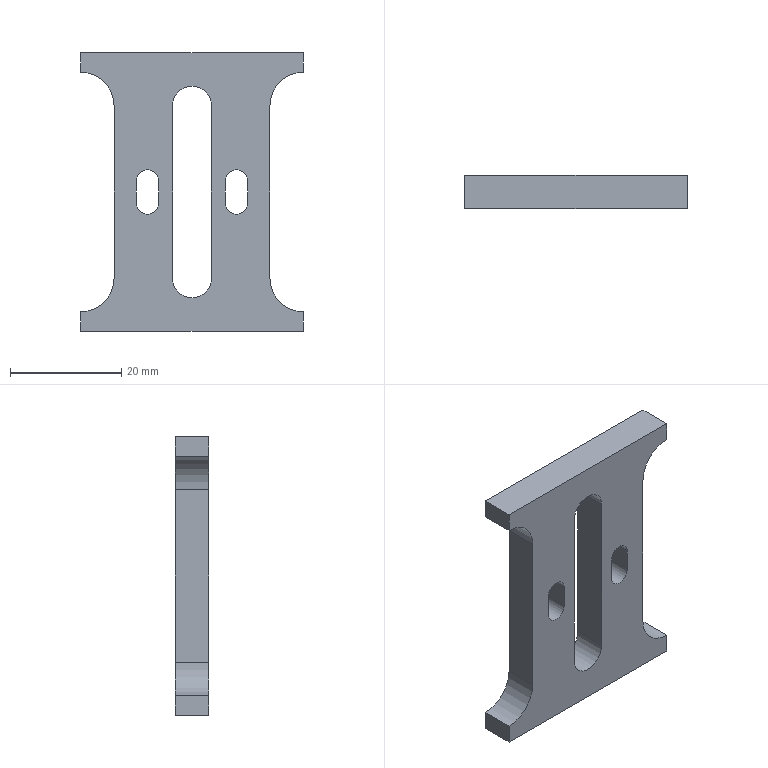Component | NX | SLIDE_PLATE_1 | 1 solid | 26 faces | volume 7214 mm3 | plane 16 | cylinder 10 | commonest cylinder face diameters 12 x4 4 x4 7 x2